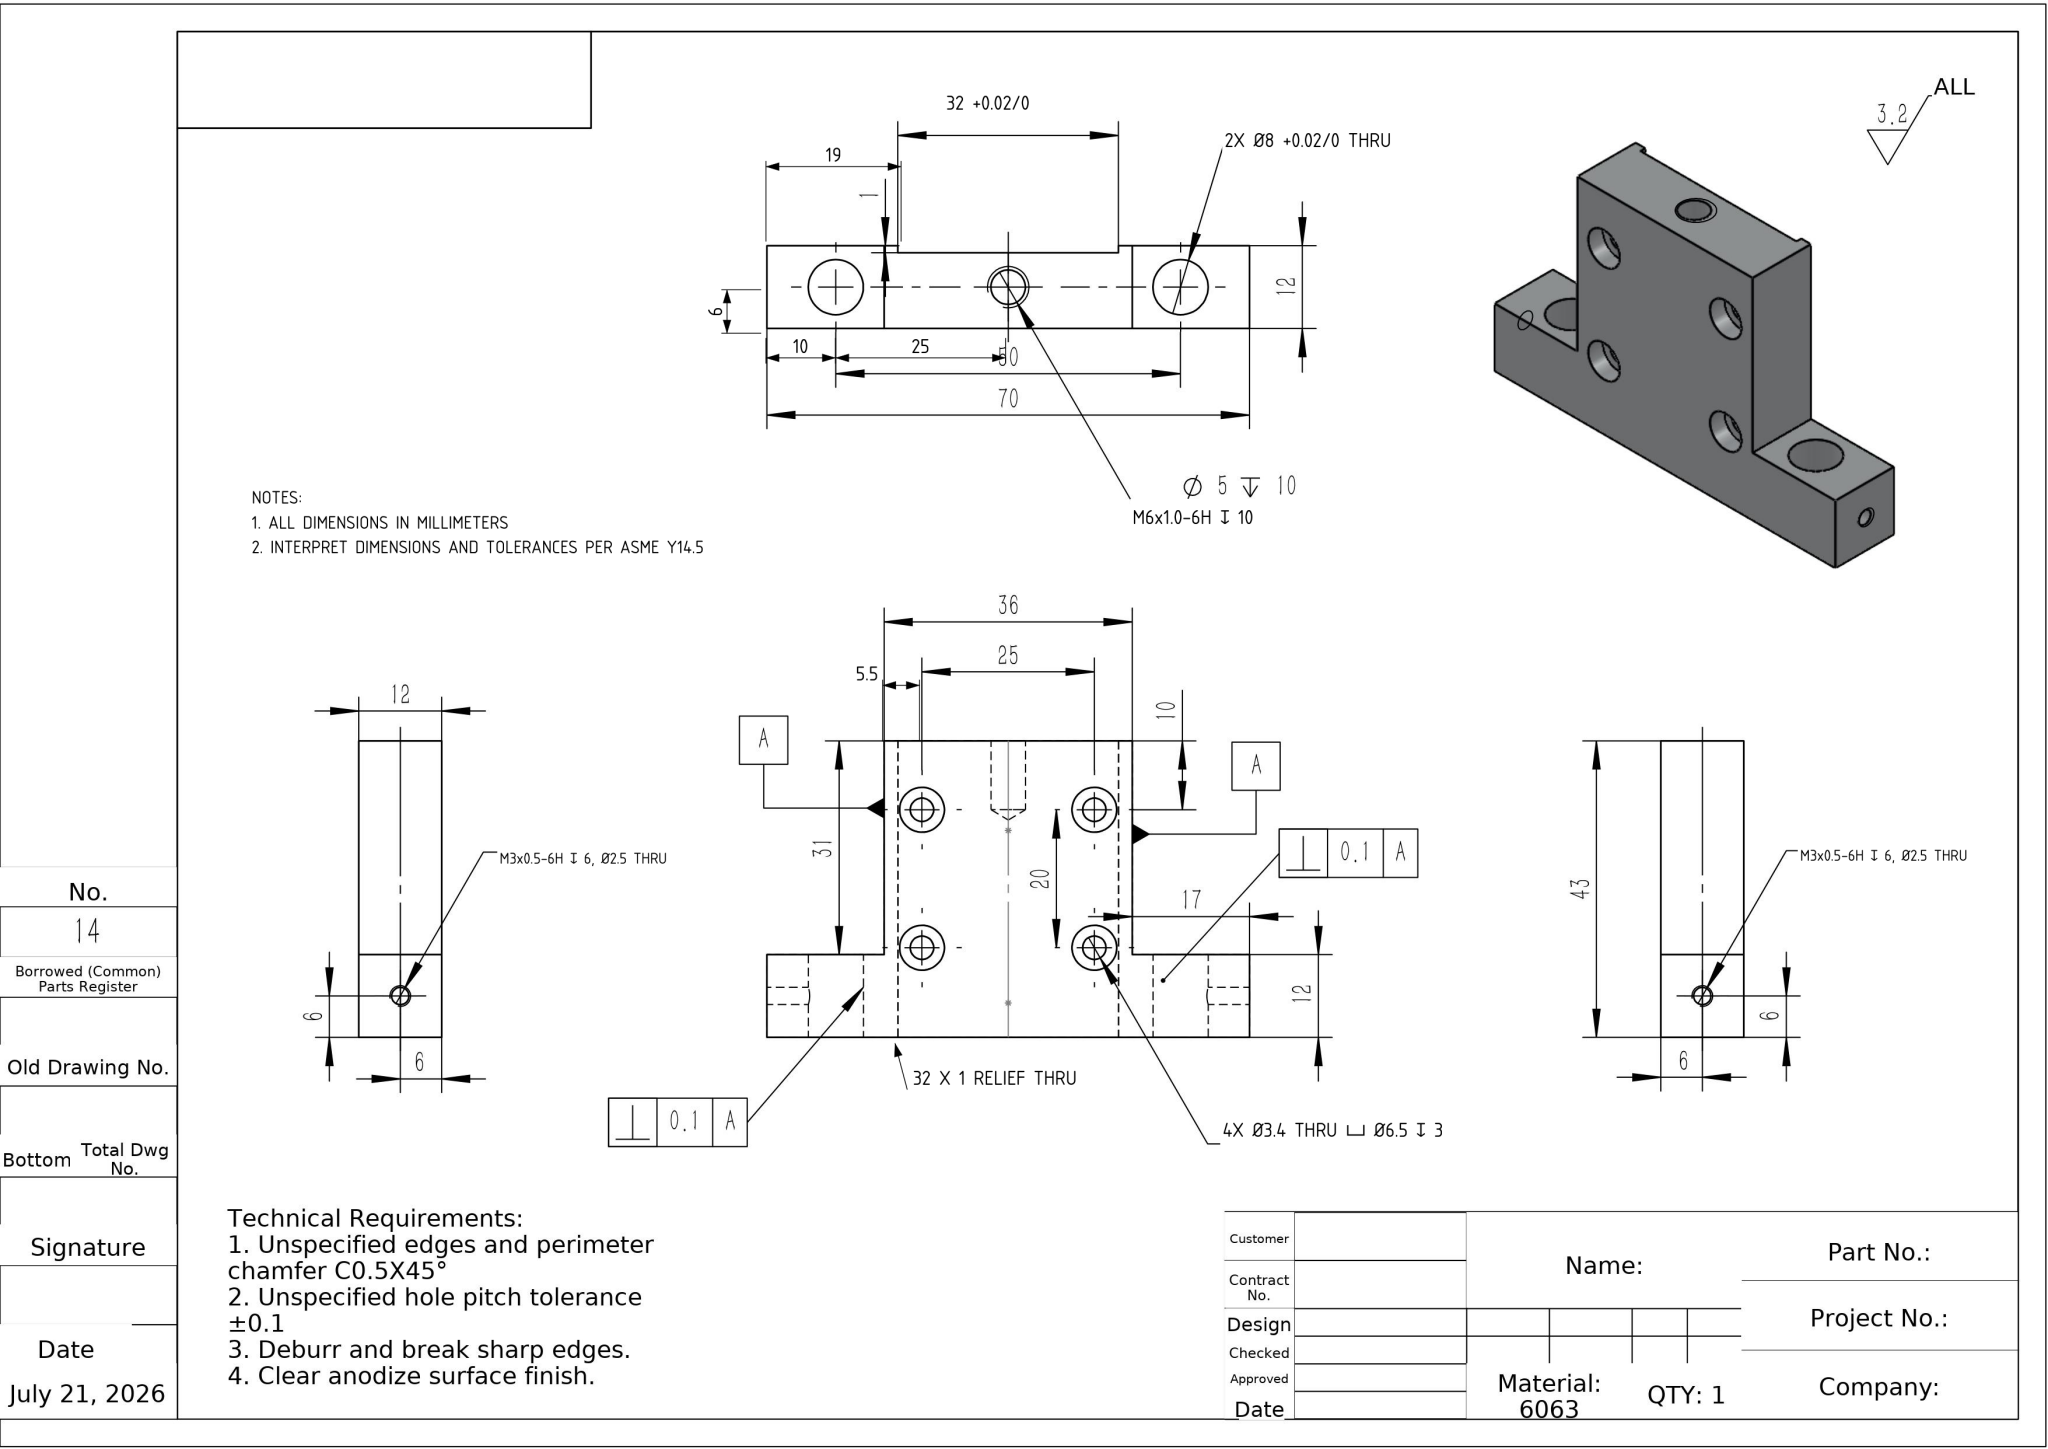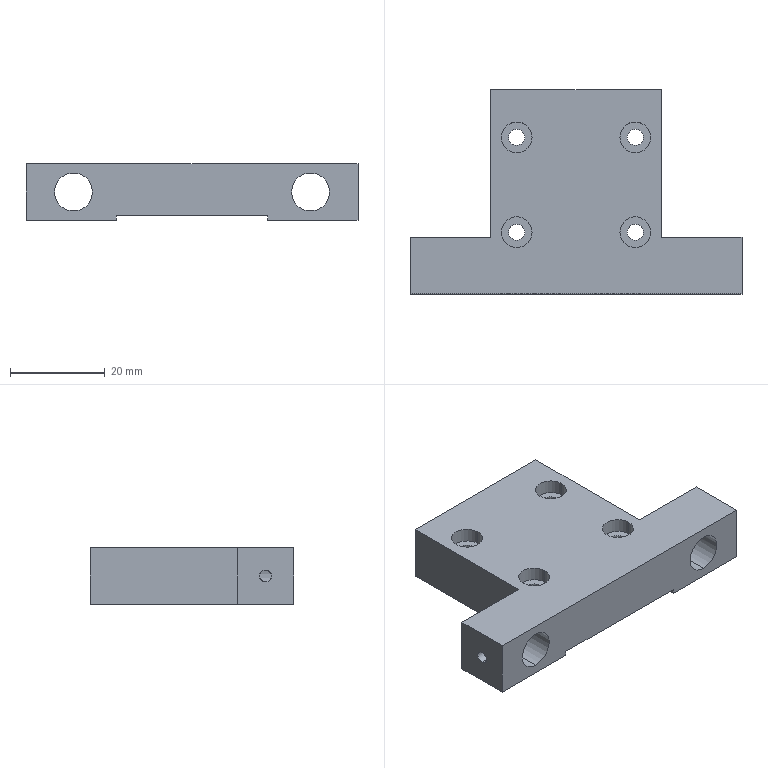Part | NX | mm | 1 solid | 46 faces | box 70 x 43 x 12 mm | volume 19935 mm3 | cylinder 26 | plane 18 | cone 2 | commonest cylinder face diameters 6.5 x8 3.4 x8 2.5 x4 8 x4 5 x2